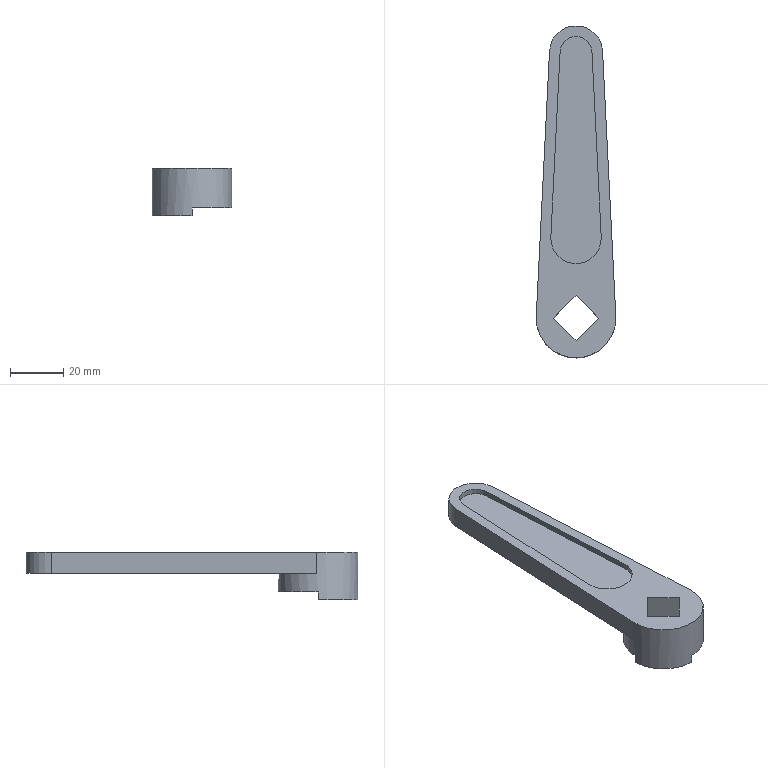Component | NX | WRENCH | 1 solid | 24 faces | volume 22181 mm3 | plane 18 | cylinder 6 | commonest cylinder face diameters 19 x2 12 x2 30 x1 20 x1